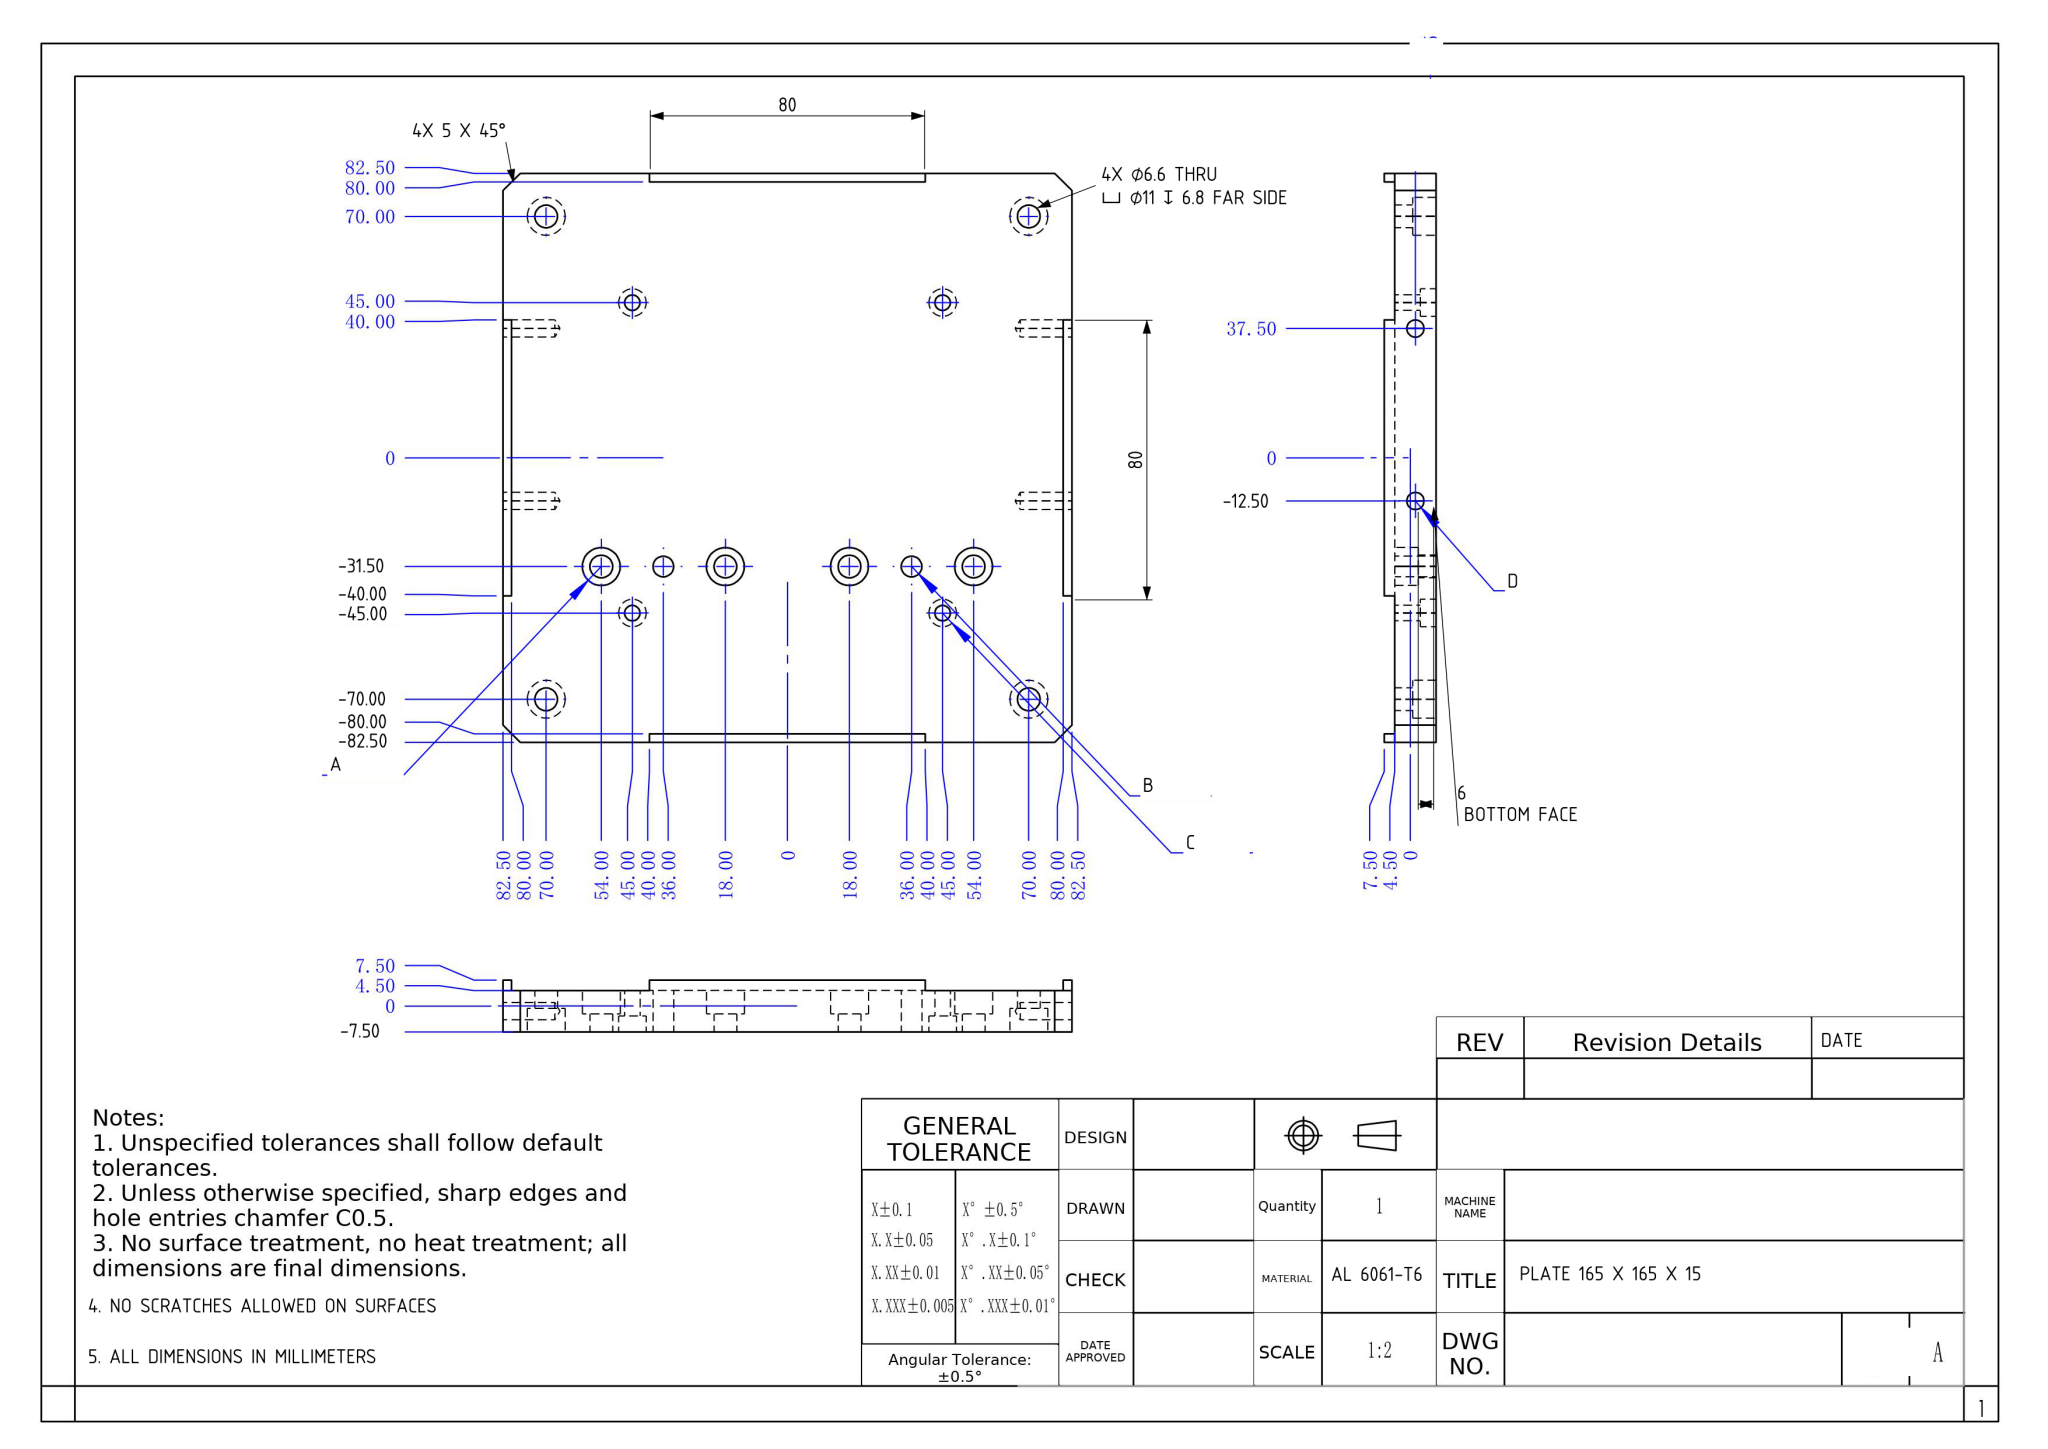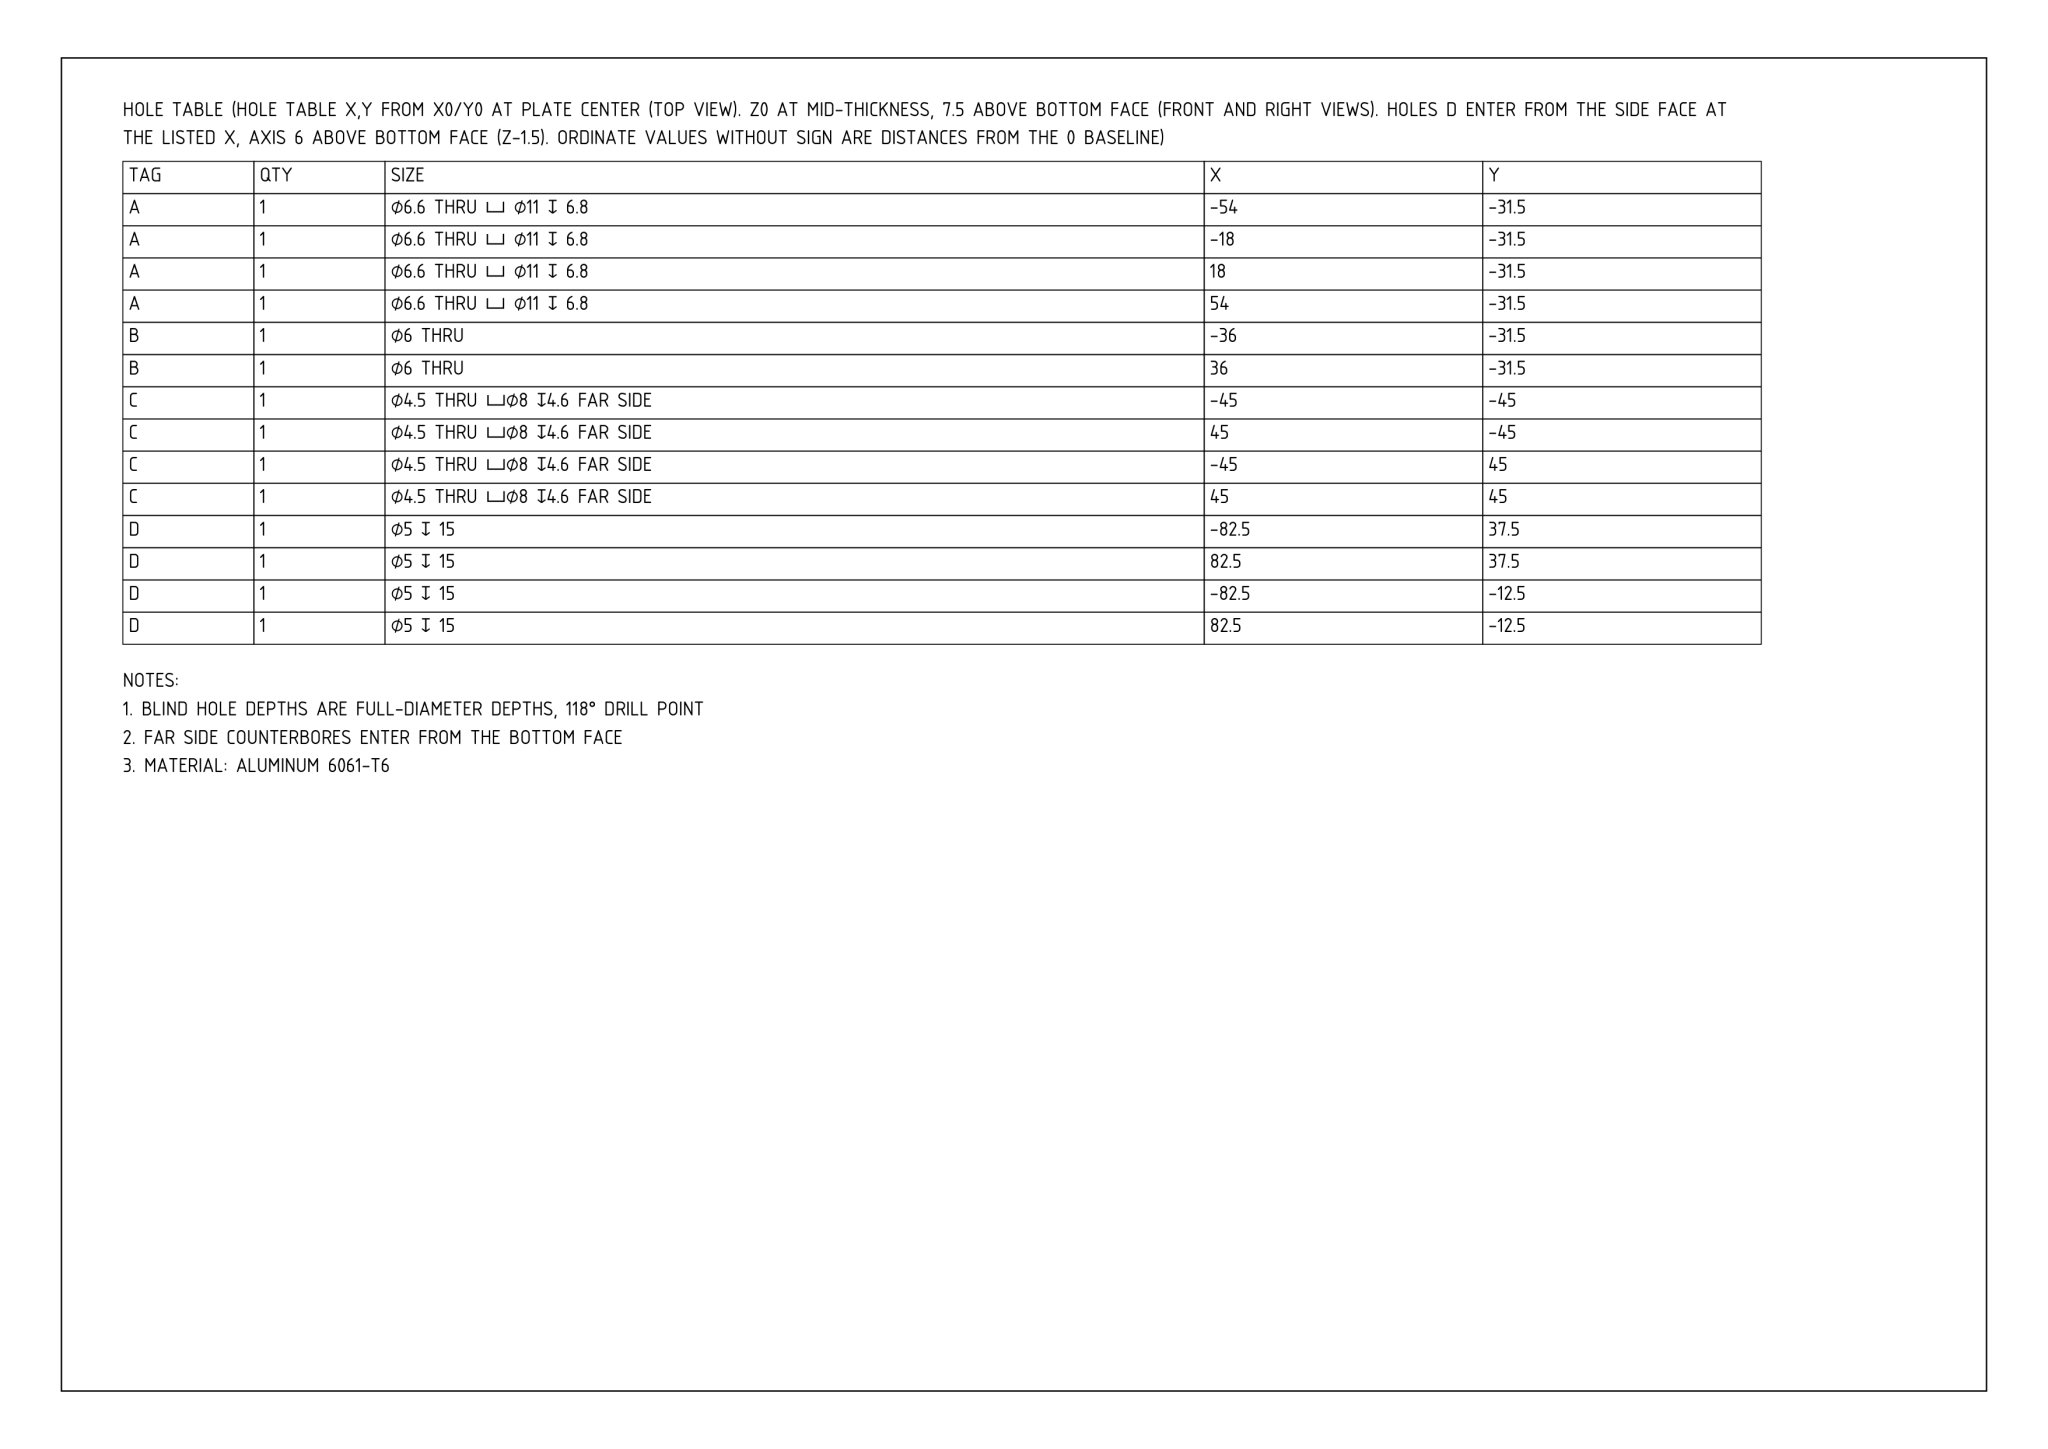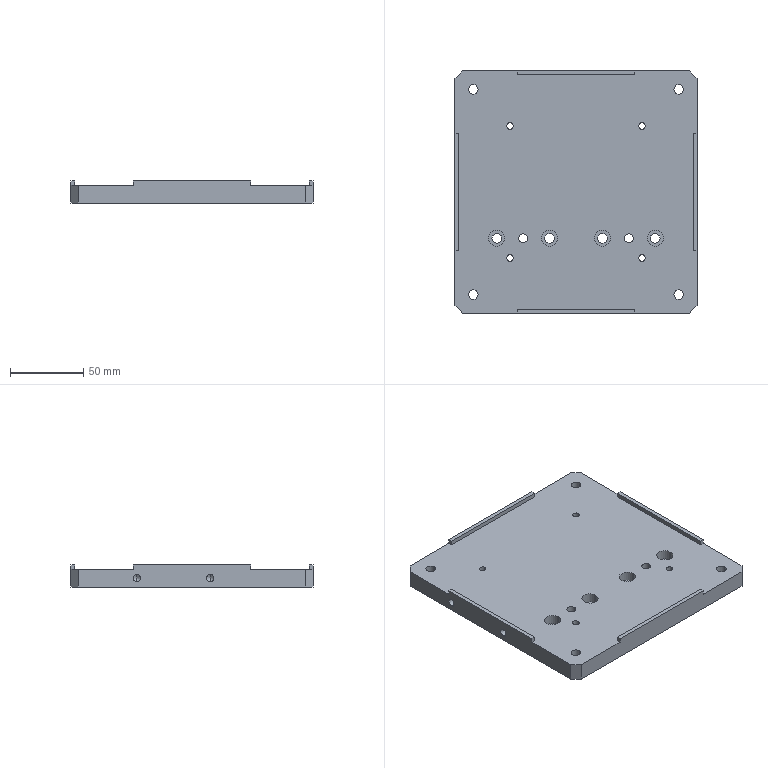Part | NX | mm | 1 solid | 106 faces | box 165 x 165 x 15 mm | volume 318615 mm3 | cylinder 60 | plane 38 | cone 8 | commonest cylinder face diameters 11 x16 6.6 x16 5 x8 8 x8 4.5 x8 6 x4